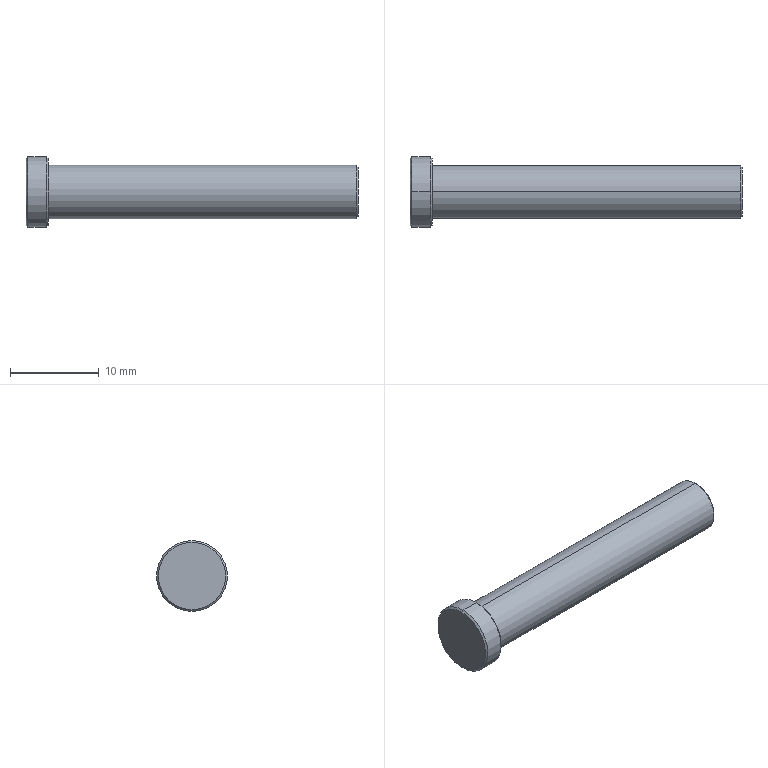Component | SolidWorks | RotatingShaft-1 | 1 solid | 13 faces | box 37.5 x 8 x 8 mm | volume 1114 mm3 | cone 6 | cylinder 4 | plane 3 | commonest cylinder face diameters 6 x2 8 x2 | material 45
build123d program:
from build123d import *

# Parameters (mm, degrees)
CHAMFER1_SIZE = 0.2


with BuildPart() as part:
    # Sketch1 → Revolve1 (revolve)
    with BuildSketch(Plane.XY, mode=Mode.PRIVATE) as revolve1_sk:
        Polygon((0, 0), (0, 4), (2.5, 4), (2.5, 3), (37.5, 3), (37.5, 0), align=None)
    revolve(revolve1_sk.sketch.rotate(Axis((0, 0, 0), (1, 0, 0)), 90), axis=Axis((0, 0, 0), (1, 0, 0)))

    # Chamfer1
    chamfer1_edges = [part.edges().sort_by_distance(p)[0] for p in [
        (37.5, 0, -3),
        (2.5, 0, -4),
        (0, 0, -4),
    ]]
    chamfer(chamfer1_edges, length=CHAMFER1_SIZE)


solid = part.part

# Placed as in the assembly
solid = solid.moved(Location((-388.859, 39.915, 1037.377), (0, 0, 0)))
STEP:
#1=CARTESIAN_POINT('',(-15.309,1.571,40.991));
#2=VERTEX_POINT('',#1);
#3=CARTESIAN_POINT('',(-15.309,1.571,40.692));
#4=VERTEX_POINT('',#3);
#5=CARTESIAN_POINT('',(-15.309,1.571,40.842));
#6=DIRECTION('',(-1.,0.,0.));
#7=DIRECTION('',(0.,0.,-1.));
#8=AXIS2_PLACEMENT_3D('',#5,#6,#7);
#9=CIRCLE('',#8,0.1496);
#10=EDGE_CURVE('',#2,#4,#9,.T.);
#11=ORIENTED_EDGE('',*,*,#10,.F.);
#12=CARTESIAN_POINT('',(-15.302,1.571,40.999));
#13=VERTEX_POINT('',#12);
#14=CARTESIAN_POINT('',(-15.309,1.571,40.991));
#15=DIRECTION('',(0.7071,0.,0.7071));
#16=VECTOR('',#15,39.37);
#17=LINE('',#14,#16);
#18=EDGE_CURVE('',#2,#13,#17,.T.);
#19=ORIENTED_EDGE('',*,*,#18,.T.);
#20=CARTESIAN_POINT('',(-15.302,1.571,40.684));
#21=VERTEX_POINT('',#20);
#22=CARTESIAN_POINT('',(-15.302,1.571,40.842));
#23=DIRECTION('',(1.,0.,0.));
#24=DIRECTION('',(0.,0.,-1.));
#25=AXIS2_PLACEMENT_3D('',#22,#23,#24);
#26=CIRCLE('',#25,0.1575);
#27=EDGE_CURVE('',#21,#13,#26,.T.);
#28=ORIENTED_EDGE('',*,*,#27,.F.);
#29=CARTESIAN_POINT('',(-15.309,1.571,40.692));
#30=DIRECTION('',(0.7071,0.,-0.7071));
#31=VECTOR('',#30,39.37);
#32=LINE('',#29,#31);
#33=EDGE_CURVE('',#4,#21,#32,.T.);
#34=ORIENTED_EDGE('',*,*,#33,.F.);
#35=EDGE_LOOP('',(#11,#19,#28,#34));
#36=FACE_OUTER_BOUND('',#35,.T.);
#37=CARTESIAN_POINT('',(-15.309,1.571,40.842));
#38=DIRECTION('',(1.,0.,0.));
#39=DIRECTION('',(0.,0.,-1.));
#40=AXIS2_PLACEMENT_3D('',#37,#38,#39);
#41=CONICAL_SURFACE('',#40,0.1496,0.7854);
#42=ADVANCED_FACE('',(#36),#41,.T.);
#43=CARTESIAN_POINT('',(-15.211,1.571,40.692));
#44=VERTEX_POINT('',#43);
#45=CARTESIAN_POINT('',(-15.211,1.571,40.991));
#46=VERTEX_POINT('',#45);
#47=CARTESIAN_POINT('',(-15.211,1.571,40.842));
#48=DIRECTION('',(1.,0.,0.));
#49=DIRECTION('',(0.,0.,1.));
#50=AXIS2_PLACEMENT_3D('',#47,#48,#49);
#51=CIRCLE('',#50,0.1496);
#52=EDGE_CURVE('',#44,#46,#51,.T.);
#53=ORIENTED_EDGE('',*,*,#52,.F.);
#54=CARTESIAN_POINT('',(-15.219,1.571,40.684));
#55=VERTEX_POINT('',#54);
#56=CARTESIAN_POINT('',(-15.219,1.571,40.684));
#57=DIRECTION('',(-0.7071,0.,-0.7071));
#58=VECTOR('',#57,39.37);
#59=LINE('',#56,#58);
#60=EDGE_CURVE('',#44,#55,#59,.T.);
#61=ORIENTED_EDGE('',*,*,#60,.T.);
#62=CARTESIAN_POINT('',(-15.219,1.571,40.999));
#63=VERTEX_POINT('',#62);
#64=CARTESIAN_POINT('',(-15.219,1.571,40.842));
#65=DIRECTION('',(-1.,0.,0.));
#66=DIRECTION('',(0.,0.,1.));
#67=AXIS2_PLACEMENT_3D('',#64,#65,#66);
#68=CIRCLE('',#67,0.1575);
#69=EDGE_CURVE('',#63,#55,#68,.T.);
#70=ORIENTED_EDGE('',*,*,#69,.F.);
#71=CARTESIAN_POINT('',(-15.219,1.571,40.999));
#72=DIRECTION('',(-0.7071,0.,0.7071));
#73=VECTOR('',#72,39.37);
#74=LINE('',#71,#73);
#75=EDGE_CURVE('',#46,#63,#74,.T.);
#76=ORIENTED_EDGE('',*,*,#75,.F.);
#77=EDGE_LOOP('',(#53,#61,#70,#76));
#78=FACE_OUTER_BOUND('',#77,.T.);
#79=CARTESIAN_POINT('',(-15.219,1.571,40.842));
#80=DIRECTION('',(-1.,0.,0.));
#81=DIRECTION('',(0.,0.,1.));
#82=AXIS2_PLACEMENT_3D('',#79,#80,#81);
#83=CONICAL_SURFACE('',#82,0.1575,0.7854);
#84=ADVANCED_FACE('',(#78),#83,.T.);
#85=CARTESIAN_POINT('',(-13.833,1.571,40.731));
#86=VERTEX_POINT('',#85);
#87=CARTESIAN_POINT('',(-13.833,1.571,40.952));
#88=VERTEX_POINT('',#87);
#89=CARTESIAN_POINT('',(-13.833,1.571,40.842));
#90=DIRECTION('',(1.,0.,0.));
#91=DIRECTION('',(0.,0.,1.));
#92=AXIS2_PLACEMENT_3D('',#89,#90,#91);
#93=CIRCLE('',#92,0.1102);
#94=EDGE_CURVE('',#86,#88,#93,.T.);
#95=ORIENTED_EDGE('',*,*,#94,.F.);
#96=CARTESIAN_POINT('',(-13.841,1.571,40.724));
#97=VERTEX_POINT('',#96);
#98=CARTESIAN_POINT('',(-13.841,1.571,40.724));
#99=DIRECTION('',(-0.7071,0.,-0.7071));
#100=VECTOR('',#99,39.37);
#101=LINE('',#98,#100);
#102=EDGE_CURVE('',#86,#97,#101,.T.);
#103=ORIENTED_EDGE('',*,*,#102,.T.);
#104=CARTESIAN_POINT('',(-13.841,1.571,40.96));
#105=VERTEX_POINT('',#104);
#106=CARTESIAN_POINT('',(-13.841,1.571,40.842));
#107=DIRECTION('',(-1.,0.,0.));
#108=DIRECTION('',(0.,0.,1.));
#109=AXIS2_PLACEMENT_3D('',#106,#107,#108);
#110=CIRCLE('',#109,0.1181);
#111=EDGE_CURVE('',#105,#97,#110,.T.);
#112=ORIENTED_EDGE('',*,*,#111,.F.);
#113=CARTESIAN_POINT('',(-13.841,1.571,40.96));
#114=DIRECTION('',(-0.7071,0.,0.7071));
#115=VECTOR('',#114,39.37);
#116=LINE('',#113,#115);
#117=EDGE_CURVE('',#88,#105,#116,.T.);
#118=ORIENTED_EDGE('',*,*,#117,.F.);
#119=EDGE_LOOP('',(#95,#103,#112,#118));
#120=FACE_OUTER_BOUND('',#119,.T.);
#121=CARTESIAN_POINT('',(-13.841,1.571,40.842));
#122=DIRECTION('',(-1.,0.,0.));
#123=DIRECTION('',(0.,0.,1.));
#124=AXIS2_PLACEMENT_3D('',#121,#122,#123);
#125=CONICAL_SURFACE('',#124,0.1181,0.7854);
#126=ADVANCED_FACE('',(#120),#125,.T.);
#127=ORIENTED_EDGE('',*,*,#111,.T.);
#128=CARTESIAN_POINT('',(-15.211,1.571,40.724));
#129=VERTEX_POINT('',#128);
#130=CARTESIAN_POINT('',(-15.309,1.571,40.724));
#131=DIRECTION('',(-1.,0.,0.));
#132=VECTOR('',#131,39.37);
#133=LINE('',#130,#132);
#134=EDGE_CURVE('',#97,#129,#133,.T.);
#135=ORIENTED_EDGE('',*,*,#134,.T.);
#136=CARTESIAN_POINT('',(-15.211,1.571,40.96));
#137=VERTEX_POINT('',#136);
#138=CARTESIAN_POINT('',(-15.211,1.571,40.842));
#139=DIRECTION('',(-1.,0.,0.));
#140=DIRECTION('',(0.,0.,1.));
#141=AXIS2_PLACEMENT_3D('',#138,#139,#140);
#142=CIRCLE('',#141,0.1181);
#143=EDGE_CURVE('',#137,#129,#142,.T.);
#144=ORIENTED_EDGE('',*,*,#143,.F.);
#145=CARTESIAN_POINT('',(-15.309,1.571,40.96));
#146=DIRECTION('',(-1.,0.,0.));
#147=VECTOR('',#146,39.37);
#148=LINE('',#145,#147);
#149=EDGE_CURVE('',#105,#137,#148,.T.);
#150=ORIENTED_EDGE('',*,*,#149,.F.);
#151=EDGE_LOOP('',(#127,#135,#144,#150));
#152=FACE_OUTER_BOUND('',#151,.T.);
#153=CARTESIAN_POINT('',(-15.309,1.571,40.842));
#154=DIRECTION('',(-1.,0.,0.));
#155=DIRECTION('',(0.,0.,1.));
#156=AXIS2_PLACEMENT_3D('',#153,#154,#155);
#157=CYLINDRICAL_SURFACE('',#156,0.1181);
#158=ADVANCED_FACE('',(#152),#157,.T.);
#159=ORIENTED_EDGE('',*,*,#69,.T.);
#160=CARTESIAN_POINT('',(-15.309,1.571,40.684));
#161=DIRECTION('',(-1.,0.,0.));
#162=VECTOR('',#161,39.37);
#163=LINE('',#160,#162);
#164=EDGE_CURVE('',#55,#21,#163,.T.);
#165=ORIENTED_EDGE('',*,*,#164,.T.);
#166=ORIENTED_EDGE('',*,*,#27,.T.);
#167=CARTESIAN_POINT('',(-15.309,1.571,40.999));
#168=DIRECTION('',(-1.,0.,0.));
#169=VECTOR('',#168,39.37);
#170=LINE('',#167,#169);
#171=EDGE_CURVE('',#63,#13,#170,.T.);
#172=ORIENTED_EDGE('',*,*,#171,.F.);
#173=EDGE_LOOP('',(#159,#165,#166,#172));
#174=FACE_OUTER_BOUND('',#173,.T.);
#175=CARTESIAN_POINT('',(-15.309,1.571,40.842));
#176=DIRECTION('',(-1.,0.,0.));
#177=DIRECTION('',(0.,0.,1.));
#178=AXIS2_PLACEMENT_3D('',#175,#176,#177);
#179=CYLINDRICAL_SURFACE('',#178,0.1575);
#180=ADVANCED_FACE('',(#174),#179,.T.);
#181=CARTESIAN_POINT('',(-15.309,1.571,40.842));
#182=DIRECTION('',(-1.,0.,0.));
#183=DIRECTION('',(0.,0.,-1.));
#184=AXIS2_PLACEMENT_3D('',#181,#182,#183);
#185=CIRCLE('',#184,0.1496);
#186=EDGE_CURVE('',#4,#2,#185,.T.);
#187=ORIENTED_EDGE('',*,*,#186,.T.);
#188=ORIENTED_EDGE('',*,*,#10,.T.);
#189=EDGE_LOOP('',(#187,#188));
#190=FACE_OUTER_BOUND('',#189,.T.);
#191=CARTESIAN_POINT('',(-15.309,1.571,40.842));
#192=DIRECTION('',(1.,0.,0.));
#193=DIRECTION('',(0.,0.,-1.));
#194=AXIS2_PLACEMENT_3D('',#191,#192,#193);
#195=PLANE('',#194);
#196=ADVANCED_FACE('',(#190),#195,.F.);
#197=ORIENTED_EDGE('',*,*,#164,.F.);
#198=CARTESIAN_POINT('',(-15.219,1.571,40.842));
#199=DIRECTION('',(-1.,0.,0.));
#200=DIRECTION('',(0.,0.,1.));
#201=AXIS2_PLACEMENT_3D('',#198,#199,#200);
#202=CIRCLE('',#201,0.1575);
#203=EDGE_CURVE('',#55,#63,#202,.T.);
#204=ORIENTED_EDGE('',*,*,#203,.T.);
#205=ORIENTED_EDGE('',*,*,#171,.T.);
#206=CARTESIAN_POINT('',(-15.302,1.571,40.842));
#207=DIRECTION('',(1.,0.,0.));
#208=DIRECTION('',(0.,0.,-1.));
#209=AXIS2_PLACEMENT_3D('',#206,#207,#208);
#210=CIRCLE('',#209,0.1575);
#211=EDGE_CURVE('',#13,#21,#210,.T.);
#212=ORIENTED_EDGE('',*,*,#211,.T.);
#213=EDGE_LOOP('',(#197,#204,#205,#212));
#214=FACE_OUTER_BOUND('',#213,.T.);
#215=CARTESIAN_POINT('',(-15.309,1.571,40.842));
#216=DIRECTION('',(-1.,0.,0.));
#217=DIRECTION('',(0.,0.,1.));
#218=AXIS2_PLACEMENT_3D('',#215,#216,#217);
#219=CYLINDRICAL_SURFACE('',#218,0.1575);
#220=ADVANCED_FACE('',(#214),#219,.T.);
#221=CARTESIAN_POINT('',(-15.211,1.571,40.842));
#222=DIRECTION('',(1.,0.,0.));
#223=DIRECTION('',(0.,0.,1.));
#224=AXIS2_PLACEMENT_3D('',#221,#222,#223);
#225=CIRCLE('',#224,0.1496);
#226=EDGE_CURVE('',#46,#44,#225,.T.);
#227=ORIENTED_EDGE('',*,*,#226,.T.);
#228=ORIENTED_EDGE('',*,*,#52,.T.);
#229=EDGE_LOOP('',(#227,#228));
#230=FACE_OUTER_BOUND('',#229,.T.);
#231=ORIENTED_EDGE('',*,*,#143,.T.);
#232=CARTESIAN_POINT('',(-15.211,1.571,40.842));
#233=DIRECTION('',(-1.,0.,0.));
#234=DIRECTION('',(0.,0.,1.));
#235=AXIS2_PLACEMENT_3D('',#232,#233,#234);
#236=CIRCLE('',#235,0.1181);
#237=EDGE_CURVE('',#129,#137,#236,.T.);
#238=ORIENTED_EDGE('',*,*,#237,.T.);
#239=EDGE_LOOP('',(#231,#238));
#240=FACE_BOUND('',#239,.T.);
#241=CARTESIAN_POINT('',(-15.211,1.729,40.842));
#242=DIRECTION('',(-1.,0.,0.));
#243=DIRECTION('',(0.,0.,1.));
#244=AXIS2_PLACEMENT_3D('',#241,#242,#243);
#245=PLANE('',#244);
#246=ADVANCED_FACE('',(#230,#240),#245,.F.);
#247=ORIENTED_EDGE('',*,*,#134,.F.);
#248=CARTESIAN_POINT('',(-13.841,1.571,40.842));
#249=DIRECTION('',(-1.,0.,0.));
#250=DIRECTION('',(0.,0.,1.));
#251=AXIS2_PLACEMENT_3D('',#248,#249,#250);
#252=CIRCLE('',#251,0.1181);
#253=EDGE_CURVE('',#97,#105,#252,.T.);
#254=ORIENTED_EDGE('',*,*,#253,.T.);
#255=ORIENTED_EDGE('',*,*,#149,.T.);
#256=ORIENTED_EDGE('',*,*,#237,.F.);
#257=EDGE_LOOP('',(#247,#254,#255,#256));
#258=FACE_OUTER_BOUND('',#257,.T.);
#259=CARTESIAN_POINT('',(-15.309,1.571,40.842));
#260=DIRECTION('',(-1.,0.,0.));
#261=DIRECTION('',(0.,0.,1.));
#262=AXIS2_PLACEMENT_3D('',#259,#260,#261);
#263=CYLINDRICAL_SURFACE('',#262,0.1181);
#264=ADVANCED_FACE('',(#258),#263,.T.);
#265=CARTESIAN_POINT('',(-13.833,1.571,40.842));
#266=DIRECTION('',(1.,0.,0.));
#267=DIRECTION('',(0.,0.,1.));
#268=AXIS2_PLACEMENT_3D('',#265,#266,#267);
#269=CIRCLE('',#268,0.1102);
#270=EDGE_CURVE('',#88,#86,#269,.T.);
#271=ORIENTED_EDGE('',*,*,#270,.T.);
#272=ORIENTED_EDGE('',*,*,#94,.T.);
#273=EDGE_LOOP('',(#271,#272));
#274=FACE_OUTER_BOUND('',#273,.T.);
#275=CARTESIAN_POINT('',(-13.833,1.69,40.842));
#276=DIRECTION('',(-1.,0.,0.));
#277=DIRECTION('',(0.,0.,1.));
#278=AXIS2_PLACEMENT_3D('',#275,#276,#277);
#279=PLANE('',#278);
#280=ADVANCED_FACE('',(#274),#279,.F.);
#281=ORIENTED_EDGE('',*,*,#102,.F.);
#282=ORIENTED_EDGE('',*,*,#270,.F.);
#283=ORIENTED_EDGE('',*,*,#117,.T.);
#284=ORIENTED_EDGE('',*,*,#253,.F.);
#285=EDGE_LOOP('',(#281,#282,#283,#284));
#286=FACE_OUTER_BOUND('',#285,.T.);
#287=CARTESIAN_POINT('',(-13.841,1.571,40.842));
#288=DIRECTION('',(-1.,0.,0.));
#289=DIRECTION('',(0.,0.,1.));
#290=AXIS2_PLACEMENT_3D('',#287,#288,#289);
#291=CONICAL_SURFACE('',#290,0.1181,0.7854);
#292=ADVANCED_FACE('',(#286),#291,.T.);
#293=ORIENTED_EDGE('',*,*,#60,.F.);
#294=ORIENTED_EDGE('',*,*,#226,.F.);
#295=ORIENTED_EDGE('',*,*,#75,.T.);
#296=ORIENTED_EDGE('',*,*,#203,.F.);
#297=EDGE_LOOP('',(#293,#294,#295,#296));
#298=FACE_OUTER_BOUND('',#297,.T.);
#299=CARTESIAN_POINT('',(-15.219,1.571,40.842));
#300=DIRECTION('',(-1.,0.,0.));
#301=DIRECTION('',(0.,0.,1.));
#302=AXIS2_PLACEMENT_3D('',#299,#300,#301);
#303=CONICAL_SURFACE('',#302,0.1575,0.7854);
#304=ADVANCED_FACE('',(#298),#303,.T.);
#305=ORIENTED_EDGE('',*,*,#18,.F.);
#306=ORIENTED_EDGE('',*,*,#186,.F.);
#307=ORIENTED_EDGE('',*,*,#33,.T.);
#308=ORIENTED_EDGE('',*,*,#211,.F.);
#309=EDGE_LOOP('',(#305,#306,#307,#308));
#310=FACE_OUTER_BOUND('',#309,.T.);
#311=CARTESIAN_POINT('',(-15.309,1.571,40.842));
#312=DIRECTION('',(1.,0.,0.));
#313=DIRECTION('',(0.,0.,-1.));
#314=AXIS2_PLACEMENT_3D('',#311,#312,#313);
#315=CONICAL_SURFACE('',#314,0.1496,0.7854);
#316=ADVANCED_FACE('',(#310),#315,.T.);
#317=CLOSED_SHELL('',(#42,#84,#126,#158,#180,#196,#220,#246,#264,#280,#292,#304,#316));
#318=MANIFOLD_SOLID_BREP('',#317);
#319=CARTESIAN_POINT('',(0.,0.,0.));
#320=DIRECTION('',(0.,0.,1.));
#321=DIRECTION('',(1.,0.,0.));
#322=AXIS2_PLACEMENT_3D('',#319,#320,#321);
#323=(LENGTH_UNIT()NAMED_UNIT(*)SI_UNIT($,.METRE.));
#324=LENGTH_MEASURE_WITH_UNIT(LENGTH_MEASURE(0.0254),#323);
#325=DIMENSIONAL_EXPONENTS(1.,0.,0.,0.,0.,0.,0.);
#326=(CONVERSION_BASED_UNIT('',#324)LENGTH_UNIT()NAMED_UNIT(#325));
#327=UNCERTAINTY_MEASURE_WITH_UNIT(LENGTH_MEASURE(0.00001),#326,'','');
#328=(NAMED_UNIT(*)PLANE_ANGLE_UNIT()SI_UNIT($,.RADIAN.));
#329=(NAMED_UNIT(*)SI_UNIT($,.STERADIAN.)SOLID_ANGLE_UNIT());
#330=(GEOMETRIC_REPRESENTATION_CONTEXT(3)GLOBAL_UNCERTAINTY_ASSIGNED_CONTEXT((#327))GLOBAL_UNIT_ASSIGNED_CONTEXT((#326,#328,#329))REPRESENTATION_CONTEXT('',''));
#331=ADVANCED_BREP_SHAPE_REPRESENTATION('',(#318,#322),#330);
#332=COLOUR_RGB('',0.7922,0.8196,0.9333);
#333=FILL_AREA_STYLE_COLOUR('',#332);
#334=FILL_AREA_STYLE('',(#333));
#335=SURFACE_STYLE_FILL_AREA(#334);
#336=SURFACE_SIDE_STYLE('',(#335));
#337=SURFACE_STYLE_USAGE(.BOTH.,#336);
#338=PRESENTATION_STYLE_ASSIGNMENT((#337));
#339=STYLED_ITEM('',(#338),#318);
#340=(LENGTH_UNIT()NAMED_UNIT(*)SI_UNIT($,.METRE.));
#341=LENGTH_MEASURE_WITH_UNIT(LENGTH_MEASURE(0.0254),#340);
#342=DIMENSIONAL_EXPONENTS(1.,0.,0.,0.,0.,0.,0.);
#343=(CONVERSION_BASED_UNIT('',#341)LENGTH_UNIT()NAMED_UNIT(#342));
#344=UNCERTAINTY_MEASURE_WITH_UNIT(LENGTH_MEASURE(0.00001),#343,'','');
#345=(NAMED_UNIT(*)PLANE_ANGLE_UNIT()SI_UNIT($,.RADIAN.));
#346=(NAMED_UNIT(*)SI_UNIT($,.STERADIAN.)SOLID_ANGLE_UNIT());
#347=(GEOMETRIC_REPRESENTATION_CONTEXT(3)GLOBAL_UNCERTAINTY_ASSIGNED_CONTEXT((#344))GLOBAL_UNIT_ASSIGNED_CONTEXT((#343,#345,#346))REPRESENTATION_CONTEXT('',''));
#348=MECHANICAL_DESIGN_GEOMETRIC_PRESENTATION_REPRESENTATION('',(#339),#347);
#349=PRESENTATION_LAYER_ASSIGNMENT('','',(#339));